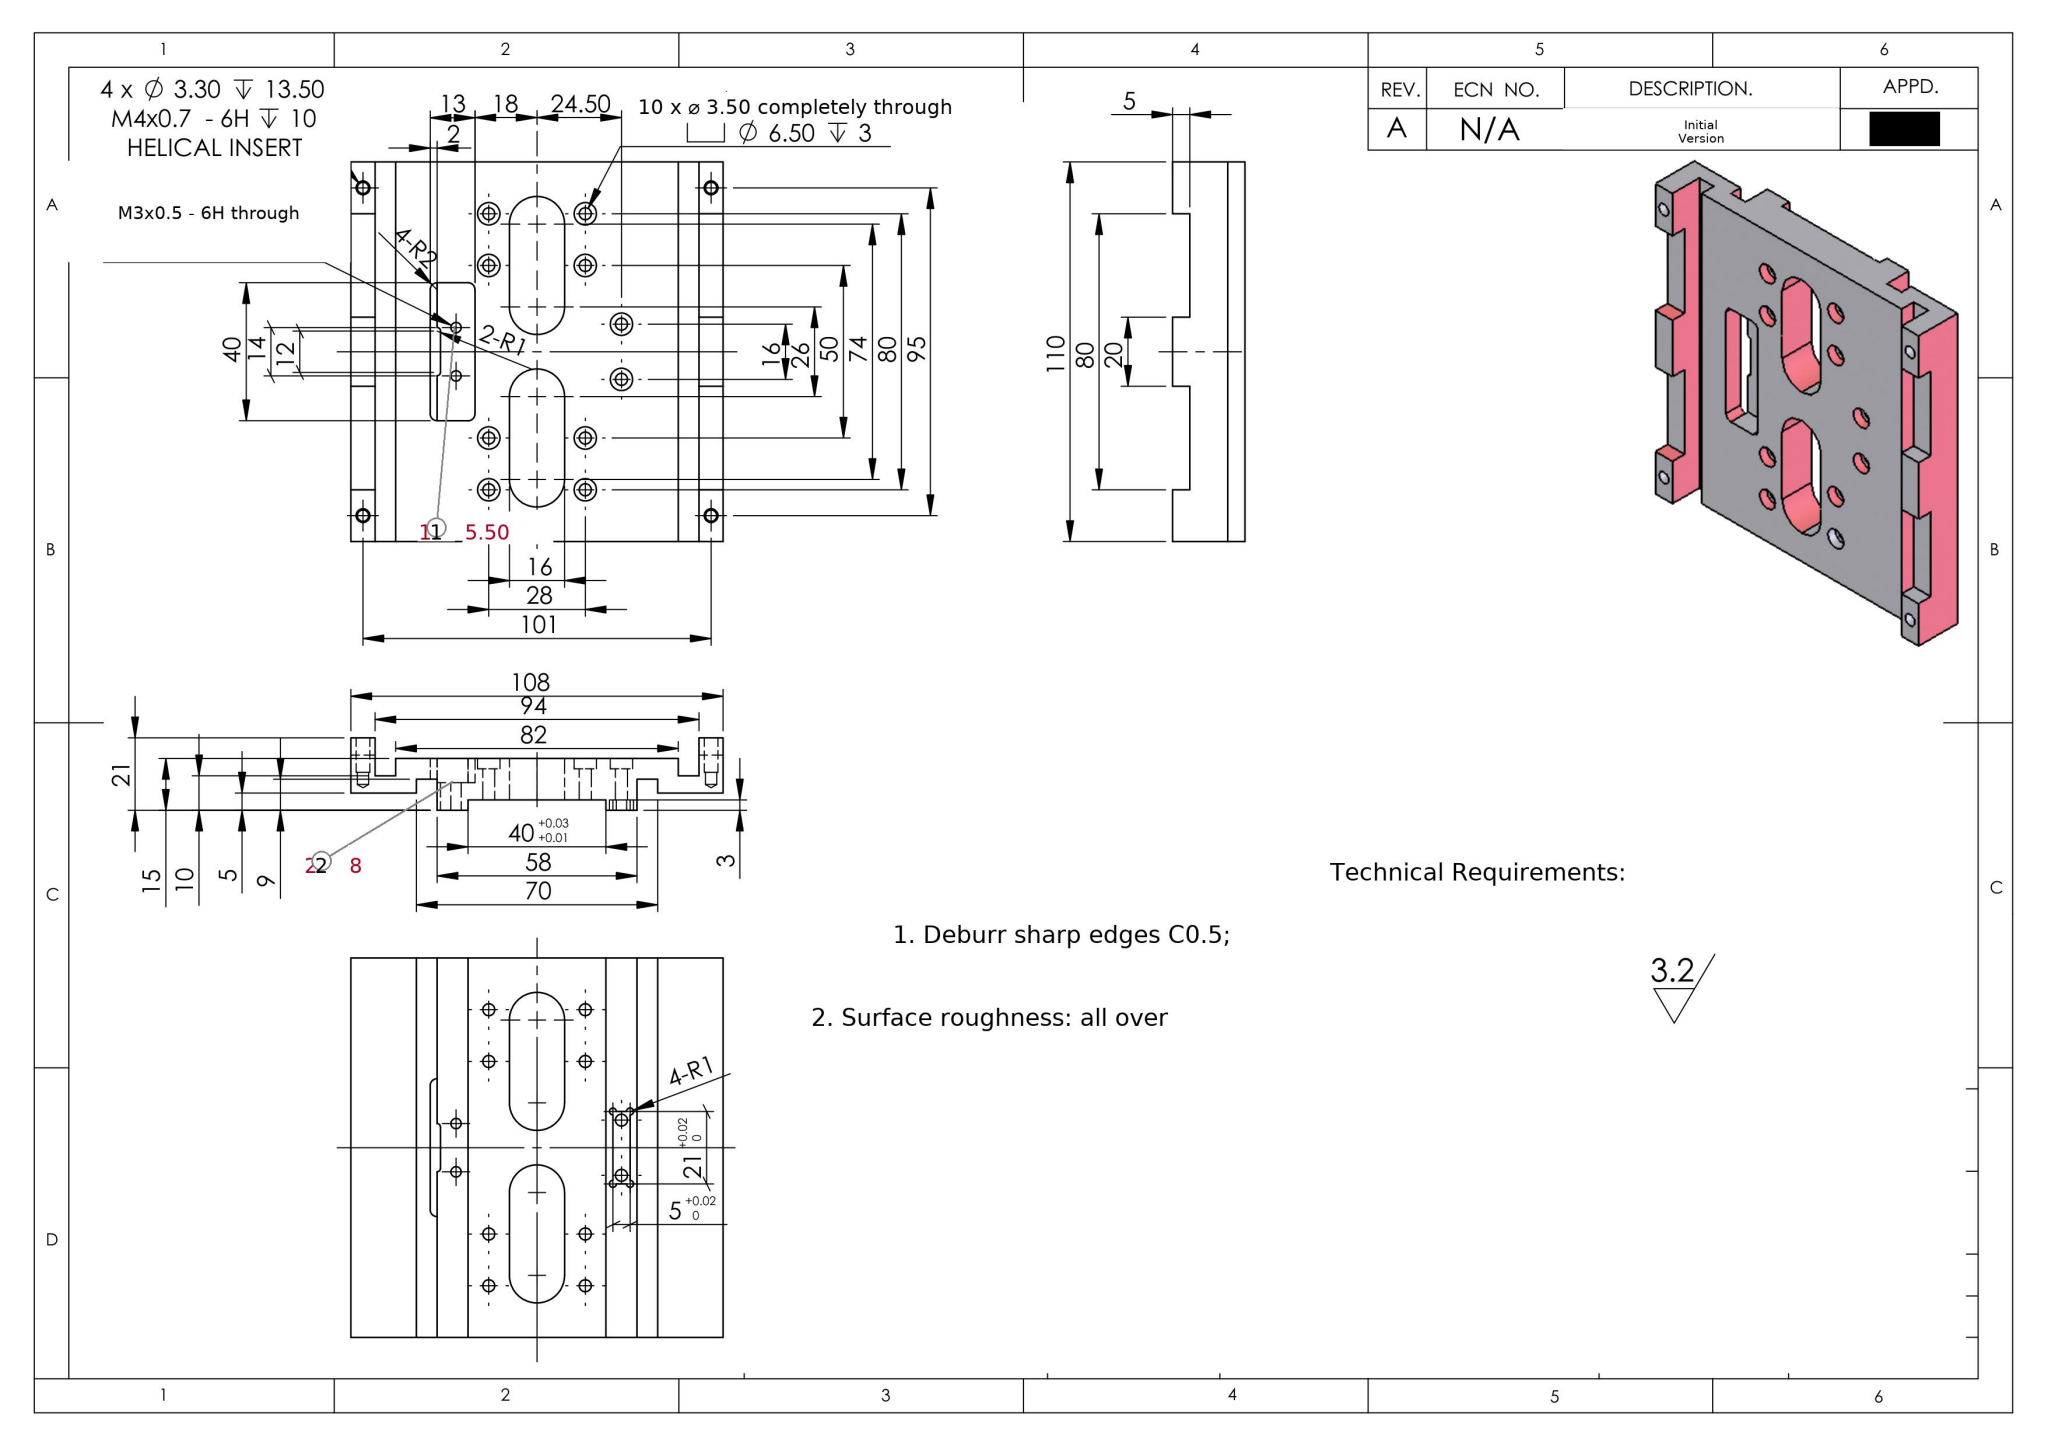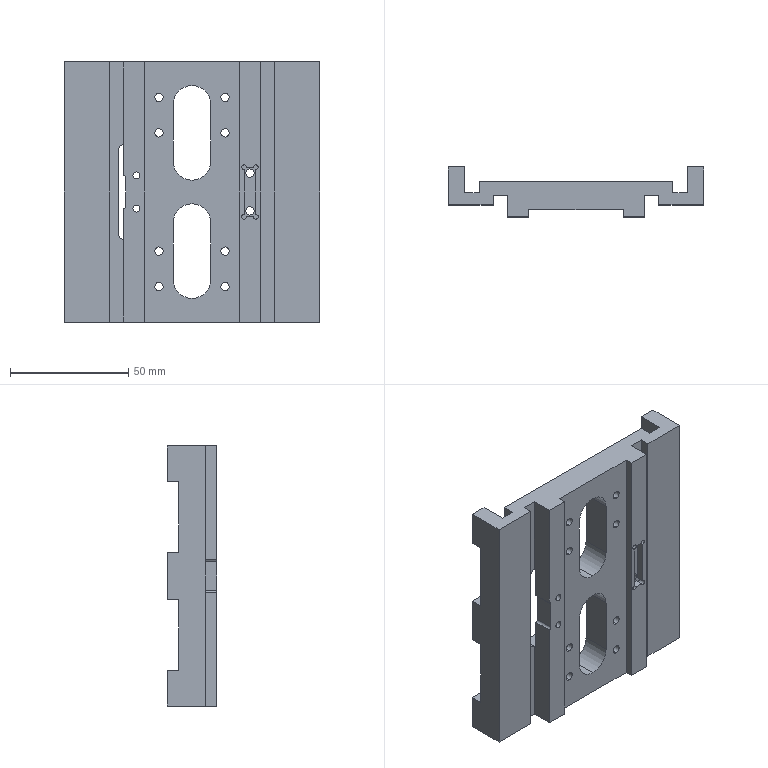Part | SolidWorks | mm | 1 solid | 160 faces | box 108 x 21 x 110 mm | volume 110021 mm3 | cylinder 80 | plane 72 | cone 8 | commonest cylinder face diameters 3.5 x20 6.5 x20 4 x12 2 x8 3.3 x8 16 x8 3 x4